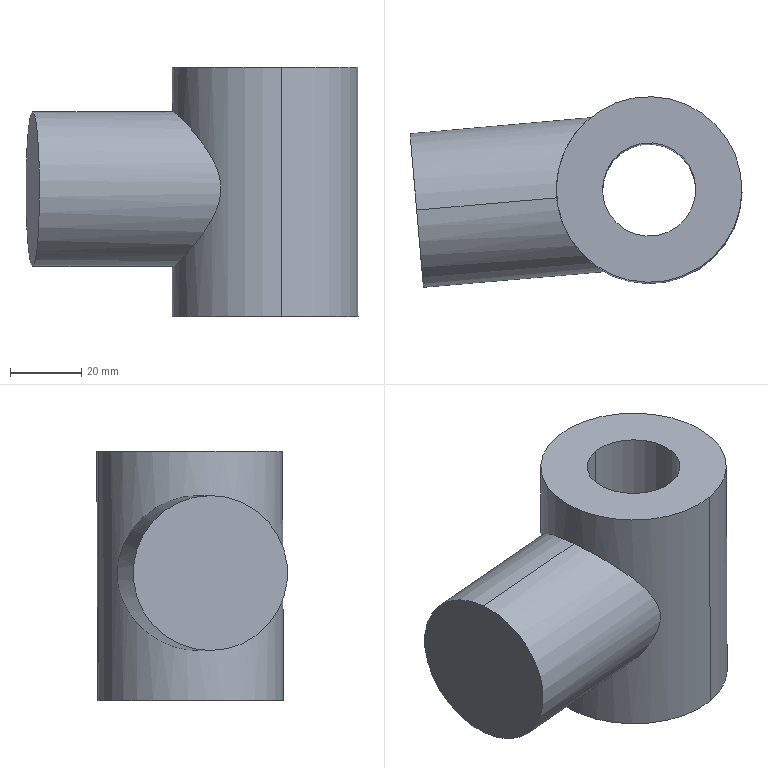Component | SolidWorks | RehabilitationChair-18-10-2 | 1 solid | 9 faces | box 93.06 x 53.47 x 70.02 mm | volume 173056 mm3 | cylinder 6 | plane 3 | commonest cylinder face diameters 43.427 x2 52.026 x2 26.129 x2
STEP:
#1=COLOUR_RGB('',0.7922,0.8196,0.9333);
#2=FILL_AREA_STYLE_COLOUR('',#1);
#3=FILL_AREA_STYLE('',(#2));
#4=SURFACE_STYLE_FILL_AREA(#3);
#5=SURFACE_SIDE_STYLE('',(#4));
#6=SURFACE_STYLE_USAGE(.BOTH.,#5);
#7=PRESENTATION_STYLE_ASSIGNMENT((#6));
#8=CARTESIAN_POINT('',(10.153,15.062,16.248));
#9=VERTEX_POINT('',#8);
#10=CARTESIAN_POINT('',(10.154,15.055,14.538));
#11=VERTEX_POINT('',#10);
#12=CARTESIAN_POINT('',(10.154,15.059,15.393));
#13=DIRECTION('',(-0.9962,-0.08716,0.));
#14=DIRECTION('',(-0.0003323,0.003798,1.));
#15=AXIS2_PLACEMENT_3D('',#12,#13,#14);
#16=CIRCLE('',#15,0.8549);
#17=EDGE_CURVE('',#9,#11,#16,.T.);
#18=ORIENTED_EDGE('',*,*,#17,.F.);
#19=CARTESIAN_POINT('',(11.698,15.197,16.248));
#20=VERTEX_POINT('',#19);
#21=CARTESIAN_POINT('',(-1.44,14.047,16.248));
#22=DIRECTION('',(0.9962,0.08716,-0.));
#23=VECTOR('',#22,39.37);
#24=LINE('',#21,#23);
#25=EDGE_CURVE('',#9,#20,#24,.T.);
#26=ORIENTED_EDGE('',*,*,#25,.T.);
#27=CARTESIAN_POINT('',(11.698,15.19,14.538));
#28=VERTEX_POINT('',#27);
#29=CARTESIAN_POINT('',(11.698,15.197,16.248));
#30=CARTESIAN_POINT('',(11.697,15.212,16.248));
#31=CARTESIAN_POINT('',(11.696,15.227,16.248));
#32=CARTESIAN_POINT('',(11.694,15.257,16.246));
#33=CARTESIAN_POINT('',(11.694,15.272,16.245));
#34=CARTESIAN_POINT('',(11.694,15.316,16.24));
#35=CARTESIAN_POINT('',(11.695,15.346,16.235));
#36=CARTESIAN_POINT('',(11.699,15.389,16.226));
#37=CARTESIAN_POINT('',(11.701,15.404,16.222));
#38=CARTESIAN_POINT('',(11.704,15.433,16.214));
#39=CARTESIAN_POINT('',(11.707,15.447,16.21));
#40=CARTESIAN_POINT('',(11.714,15.489,16.197));
#41=CARTESIAN_POINT('',(11.72,15.517,16.186));
#42=CARTESIAN_POINT('',(11.734,15.57,16.163));
#43=CARTESIAN_POINT('',(11.742,15.596,16.151));
#44=CARTESIAN_POINT('',(11.759,15.646,16.123));
#45=CARTESIAN_POINT('',(11.769,15.671,16.108));
#46=CARTESIAN_POINT('',(11.799,15.741,16.061));
#47=CARTESIAN_POINT('',(11.822,15.783,16.026));
#48=CARTESIAN_POINT('',(11.858,15.842,15.969));
#49=CARTESIAN_POINT('',(11.871,15.861,15.95));
#50=CARTESIAN_POINT('',(11.896,15.896,15.908));
#51=CARTESIAN_POINT('',(11.909,15.913,15.887));
#52=CARTESIAN_POINT('',(11.947,15.96,15.821));
#53=CARTESIAN_POINT('',(11.973,15.987,15.775));
#54=CARTESIAN_POINT('',(12.008,16.022,15.7));
#55=CARTESIAN_POINT('',(12.019,16.032,15.675));
#56=CARTESIAN_POINT('',(12.04,16.051,15.621));
#57=CARTESIAN_POINT('',(12.049,16.059,15.594));
#58=CARTESIAN_POINT('',(12.065,16.072,15.538));
#59=CARTESIAN_POINT('',(12.071,16.077,15.509));
#60=CARTESIAN_POINT('',(12.08,16.084,15.449));
#61=CARTESIAN_POINT('',(12.082,16.085,15.419));
#62=CARTESIAN_POINT('',(12.082,16.085,15.36));
#63=CARTESIAN_POINT('',(12.08,16.083,15.33));
#64=CARTESIAN_POINT('',(12.071,16.076,15.271));
#65=CARTESIAN_POINT('',(12.065,16.071,15.242));
#66=CARTESIAN_POINT('',(12.049,16.057,15.186));
#67=CARTESIAN_POINT('',(12.04,16.049,15.159));
#68=CARTESIAN_POINT('',(12.024,16.035,15.119));
#69=CARTESIAN_POINT('',(12.019,16.03,15.106));
#70=CARTESIAN_POINT('',(12.008,16.019,15.08));
#71=CARTESIAN_POINT('',(12.002,16.014,15.067));
#72=CARTESIAN_POINT('',(11.973,15.984,15.005));
#73=CARTESIAN_POINT('',(11.947,15.957,14.959));
#74=CARTESIAN_POINT('',(11.909,15.909,14.893));
#75=CARTESIAN_POINT('',(11.896,15.892,14.872));
#76=CARTESIAN_POINT('',(11.871,15.856,14.831));
#77=CARTESIAN_POINT('',(11.859,15.837,14.812));
#78=CARTESIAN_POINT('',(11.822,15.778,14.755));
#79=CARTESIAN_POINT('',(11.8,15.735,14.721));
#80=CARTESIAN_POINT('',(11.774,15.677,14.682));
#81=CARTESIAN_POINT('',(11.769,15.665,14.675));
#82=CARTESIAN_POINT('',(11.76,15.641,14.66));
#83=CARTESIAN_POINT('',(11.755,15.628,14.653));
#84=CARTESIAN_POINT('',(11.742,15.59,14.632));
#85=CARTESIAN_POINT('',(11.734,15.564,14.62));
#86=CARTESIAN_POINT('',(11.72,15.511,14.598));
#87=CARTESIAN_POINT('',(11.715,15.483,14.587));
#88=CARTESIAN_POINT('',(11.705,15.427,14.57));
#89=CARTESIAN_POINT('',(11.701,15.398,14.562));
#90=CARTESIAN_POINT('',(11.693,15.31,14.544));
#91=CARTESIAN_POINT('',(11.693,15.251,14.538));
#92=CARTESIAN_POINT('',(11.698,15.19,14.538));
#93=B_SPLINE_CURVE_WITH_KNOTS('',3,(#29,#30,#31,#32,#33,#34,#35,#36,#37,#38,#39,#40,#41,#42,#43,#44,#45,#46,#47,#48,#49,#50,#51,#52,#53,#54,#55,#56,#57,#58,#59,#60,#61,#62,#63,#64,#65,#66,#67,#68,#69,#70,#71,#72,#73,#74,#75,#76,#77,#78,#79,#80,#81,#82,#83,#84,#85,#86,#87,#88,#89,#90,#91,#92),.UNSPECIFIED.,.F.,.F.,(4,2,2,2,2,2,2,2,2,2,2,2,2,2,2,2,2,2,2,2,2,2,2,2,2,2,2,2,2,2,2,4),(0.07253,0.07367,0.0748,0.07706,0.07819,0.07933,0.08159,0.08385,0.08612,0.09065,0.09291,0.09517,0.0997,0.102,0.1042,0.1065,0.1088,0.111,0.1133,0.1155,0.1167,0.1178,0.1223,0.1246,0.1269,0.1314,0.1325,0.1337,0.1359,0.1382,0.1405,0.145),.UNSPECIFIED.);
#94=EDGE_CURVE('',#20,#28,#93,.T.);
#95=ORIENTED_EDGE('',*,*,#94,.T.);
#96=CARTESIAN_POINT('',(-1.44,14.041,14.538));
#97=DIRECTION('',(0.9962,0.08716,-0.));
#98=VECTOR('',#97,39.37);
#99=LINE('',#96,#98);
#100=EDGE_CURVE('',#11,#28,#99,.T.);
#101=ORIENTED_EDGE('',*,*,#100,.F.);
#102=EDGE_LOOP('',(#18,#26,#95,#101));
#103=FACE_OUTER_BOUND('',#102,.T.);
#104=CARTESIAN_POINT('',(-1.44,14.044,15.393));
#105=DIRECTION('',(0.9962,0.08716,-0.));
#106=DIRECTION('',(0.0003323,-0.003798,-1.));
#107=AXIS2_PLACEMENT_3D('',#104,#105,#106);
#108=CYLINDRICAL_SURFACE('',#107,0.8549);
#109=ADVANCED_FACE('',(#103),#108,.T.);
#110=CARTESIAN_POINT('',(12.897,14.269,13.99));
#111=VERTEX_POINT('',#110);
#112=CARTESIAN_POINT('',(12.541,16.286,13.982));
#113=VERTEX_POINT('',#112);
#114=CARTESIAN_POINT('',(12.719,15.278,13.986));
#115=DIRECTION('',(-0.0003323,0.003798,1.));
#116=DIRECTION('',(-0.9962,-0.08716,0.));
#117=AXIS2_PLACEMENT_3D('',#114,#115,#116);
#118=CIRCLE('',#117,1.024);
#119=EDGE_CURVE('',#111,#113,#118,.T.);
#120=ORIENTED_EDGE('',*,*,#119,.T.);
#121=CARTESIAN_POINT('',(12.54,16.297,16.731));
#122=VERTEX_POINT('',#121);
#123=CARTESIAN_POINT('',(12.541,16.283,13.195));
#124=DIRECTION('',(-0.0003323,0.003798,1.));
#125=VECTOR('',#124,39.37);
#126=LINE('',#123,#125);
#127=EDGE_CURVE('',#113,#122,#126,.T.);
#128=ORIENTED_EDGE('',*,*,#127,.T.);
#129=CARTESIAN_POINT('',(12.896,14.279,16.739));
#130=VERTEX_POINT('',#129);
#131=CARTESIAN_POINT('',(12.718,15.288,16.735));
#132=DIRECTION('',(-0.0003323,0.003798,1.));
#133=DIRECTION('',(-0.9962,-0.08716,0.));
#134=AXIS2_PLACEMENT_3D('',#131,#132,#133);
#135=CIRCLE('',#134,1.024);
#136=EDGE_CURVE('',#130,#122,#135,.T.);
#137=ORIENTED_EDGE('',*,*,#136,.F.);
#138=CARTESIAN_POINT('',(12.897,14.266,13.203));
#139=DIRECTION('',(-0.0003323,0.003798,1.));
#140=VECTOR('',#139,39.37);
#141=LINE('',#138,#140);
#142=EDGE_CURVE('',#111,#130,#141,.T.);
#143=ORIENTED_EDGE('',*,*,#142,.F.);
#144=EDGE_LOOP('',(#120,#128,#137,#143));
#145=FACE_OUTER_BOUND('',#144,.T.);
#146=CARTESIAN_POINT('',(12.719,15.275,13.199));
#147=DIRECTION('',(-0.0003323,0.003798,1.));
#148=DIRECTION('',(0.1736,-0.9848,0.003798));
#149=AXIS2_PLACEMENT_3D('',#146,#147,#148);
#150=CYLINDRICAL_SURFACE('',#149,1.024);
#151=ADVANCED_FACE('',(#145),#150,.T.);
#152=CARTESIAN_POINT('',(12.629,15.795,16.733));
#153=VERTEX_POINT('',#152);
#154=CARTESIAN_POINT('',(12.807,14.781,16.737));
#155=VERTEX_POINT('',#154);
#156=CARTESIAN_POINT('',(12.718,15.288,16.735));
#157=DIRECTION('',(-0.0003323,0.003798,1.));
#158=DIRECTION('',(0.1736,-0.9848,0.003798));
#159=AXIS2_PLACEMENT_3D('',#156,#157,#158);
#160=CIRCLE('',#159,0.5144);
#161=EDGE_CURVE('',#153,#155,#160,.T.);
#162=ORIENTED_EDGE('',*,*,#161,.T.);
#163=CARTESIAN_POINT('',(12.808,14.771,13.988));
#164=VERTEX_POINT('',#163);
#165=CARTESIAN_POINT('',(12.807,14.781,16.734));
#166=DIRECTION('',(0.0003323,-0.003798,-1.));
#167=VECTOR('',#166,39.37);
#168=LINE('',#165,#167);
#169=EDGE_CURVE('',#155,#164,#168,.T.);
#170=ORIENTED_EDGE('',*,*,#169,.T.);
#171=CARTESIAN_POINT('',(12.63,15.784,13.984));
#172=VERTEX_POINT('',#171);
#173=CARTESIAN_POINT('',(12.719,15.278,13.986));
#174=DIRECTION('',(0.0003323,-0.003798,-1.));
#175=DIRECTION('',(0.1736,-0.9848,0.003798));
#176=AXIS2_PLACEMENT_3D('',#173,#174,#175);
#177=CIRCLE('',#176,0.5144);
#178=EDGE_CURVE('',#164,#172,#177,.T.);
#179=ORIENTED_EDGE('',*,*,#178,.T.);
#180=CARTESIAN_POINT('',(12.629,15.795,16.73));
#181=DIRECTION('',(0.0003323,-0.003798,-1.));
#182=VECTOR('',#181,39.37);
#183=LINE('',#180,#182);
#184=EDGE_CURVE('',#153,#172,#183,.T.);
#185=ORIENTED_EDGE('',*,*,#184,.F.);
#186=EDGE_LOOP('',(#162,#170,#179,#185));
#187=FACE_OUTER_BOUND('',#186,.T.);
#188=CARTESIAN_POINT('',(12.718,15.288,16.732));
#189=DIRECTION('',(0.0003323,-0.003798,-1.));
#190=DIRECTION('',(-0.1736,0.9848,-0.003798));
#191=AXIS2_PLACEMENT_3D('',#188,#189,#190);
#192=CYLINDRICAL_SURFACE('',#191,0.5144);
#193=ADVANCED_FACE('',(#187),#192,.F.);
#194=ORIENTED_EDGE('',*,*,#119,.F.);
#195=CARTESIAN_POINT('',(12.719,15.278,13.986));
#196=DIRECTION('',(-0.0003323,0.003798,1.));
#197=DIRECTION('',(-0.9962,-0.08716,0.));
#198=AXIS2_PLACEMENT_3D('',#195,#196,#197);
#199=CIRCLE('',#198,1.024);
#200=EDGE_CURVE('',#113,#111,#199,.T.);
#201=ORIENTED_EDGE('',*,*,#200,.F.);
#202=EDGE_LOOP('',(#194,#201));
#203=FACE_OUTER_BOUND('',#202,.T.);
#204=CARTESIAN_POINT('',(12.719,15.278,13.986));
#205=DIRECTION('',(0.0003323,-0.003798,-1.));
#206=DIRECTION('',(0.1736,-0.9848,0.003798));
#207=AXIS2_PLACEMENT_3D('',#204,#205,#206);
#208=CIRCLE('',#207,0.5144);
#209=EDGE_CURVE('',#172,#164,#208,.T.);
#210=ORIENTED_EDGE('',*,*,#209,.F.);
#211=ORIENTED_EDGE('',*,*,#178,.F.);
#212=EDGE_LOOP('',(#210,#211));
#213=FACE_BOUND('',#212,.T.);
#214=CARTESIAN_POINT('',(13.727,15.455,13.986));
#215=DIRECTION('',(-0.0003323,0.003798,1.));
#216=DIRECTION('',(0.1736,-0.9848,0.003798));
#217=AXIS2_PLACEMENT_3D('',#214,#215,#216);
#218=PLANE('',#217);
#219=ADVANCED_FACE('',(#203,#213),#218,.F.);
#220=CARTESIAN_POINT('',(10.154,15.059,15.393));
#221=DIRECTION('',(-0.9962,-0.08716,0.));
#222=DIRECTION('',(-0.0003323,0.003798,1.));
#223=AXIS2_PLACEMENT_3D('',#220,#221,#222);
#224=CIRCLE('',#223,0.8549);
#225=EDGE_CURVE('',#11,#9,#224,.T.);
#226=ORIENTED_EDGE('',*,*,#225,.T.);
#227=ORIENTED_EDGE('',*,*,#17,.T.);
#228=EDGE_LOOP('',(#226,#227));
#229=FACE_OUTER_BOUND('',#228,.T.);
#230=CARTESIAN_POINT('',(9.938,17.521,42.747));
#231=DIRECTION('',(-0.9962,-0.08716,0.));
#232=DIRECTION('',(-0.0003323,0.003798,1.));
#233=AXIS2_PLACEMENT_3D('',#230,#231,#232);
#234=PLANE('',#233);
#235=ADVANCED_FACE('',(#229),#234,.T.);
#236=ORIENTED_EDGE('',*,*,#25,.F.);
#237=ORIENTED_EDGE('',*,*,#225,.F.);
#238=ORIENTED_EDGE('',*,*,#100,.T.);
#239=CARTESIAN_POINT('',(11.698,15.19,14.538));
#240=CARTESIAN_POINT('',(11.704,15.13,14.539));
#241=CARTESIAN_POINT('',(11.714,15.072,14.545));
#242=CARTESIAN_POINT('',(11.733,15.001,14.561));
#243=CARTESIAN_POINT('',(11.737,14.987,14.564));
#244=CARTESIAN_POINT('',(11.746,14.96,14.572));
#245=CARTESIAN_POINT('',(11.75,14.946,14.576));
#246=CARTESIAN_POINT('',(11.765,14.905,14.59));
#247=CARTESIAN_POINT('',(11.776,14.879,14.6));
#248=CARTESIAN_POINT('',(11.799,14.829,14.623));
#249=CARTESIAN_POINT('',(11.811,14.805,14.635));
#250=CARTESIAN_POINT('',(11.837,14.759,14.663));
#251=CARTESIAN_POINT('',(11.851,14.736,14.678));
#252=CARTESIAN_POINT('',(11.893,14.672,14.725));
#253=CARTESIAN_POINT('',(11.923,14.634,14.76));
#254=CARTESIAN_POINT('',(11.968,14.583,14.817));
#255=CARTESIAN_POINT('',(11.984,14.567,14.836));
#256=CARTESIAN_POINT('',(12.015,14.536,14.878));
#257=CARTESIAN_POINT('',(12.031,14.522,14.899));
#258=CARTESIAN_POINT('',(12.077,14.482,14.965));
#259=CARTESIAN_POINT('',(12.106,14.46,15.011));
#260=CARTESIAN_POINT('',(12.14,14.436,15.073));
#261=CARTESIAN_POINT('',(12.147,14.432,15.086));
#262=CARTESIAN_POINT('',(12.16,14.424,15.112));
#263=CARTESIAN_POINT('',(12.166,14.42,15.125));
#264=CARTESIAN_POINT('',(12.184,14.409,15.165));
#265=CARTESIAN_POINT('',(12.194,14.402,15.193));
#266=CARTESIAN_POINT('',(12.207,14.395,15.235));
#267=CARTESIAN_POINT('',(12.211,14.393,15.249));
#268=CARTESIAN_POINT('',(12.218,14.389,15.278));
#269=CARTESIAN_POINT('',(12.221,14.387,15.293));
#270=CARTESIAN_POINT('',(12.229,14.383,15.337));
#271=CARTESIAN_POINT('',(12.231,14.382,15.367));
#272=CARTESIAN_POINT('',(12.231,14.382,15.427));
#273=CARTESIAN_POINT('',(12.229,14.384,15.456));
#274=CARTESIAN_POINT('',(12.219,14.389,15.516));
#275=CARTESIAN_POINT('',(12.211,14.394,15.545));
#276=CARTESIAN_POINT('',(12.194,14.404,15.601));
#277=CARTESIAN_POINT('',(12.183,14.41,15.628));
#278=CARTESIAN_POINT('',(12.165,14.422,15.668));
#279=CARTESIAN_POINT('',(12.159,14.426,15.681));
#280=CARTESIAN_POINT('',(12.146,14.434,15.707));
#281=CARTESIAN_POINT('',(12.14,14.439,15.719));
#282=CARTESIAN_POINT('',(12.106,14.463,15.782));
#283=CARTESIAN_POINT('',(12.076,14.486,15.828));
#284=CARTESIAN_POINT('',(12.03,14.526,15.893));
#285=CARTESIAN_POINT('',(12.014,14.541,15.914));
#286=CARTESIAN_POINT('',(11.983,14.572,15.955));
#287=CARTESIAN_POINT('',(11.968,14.588,15.975));
#288=CARTESIAN_POINT('',(11.922,14.64,16.031));
#289=CARTESIAN_POINT('',(11.892,14.678,16.066));
#290=CARTESIAN_POINT('',(11.85,14.742,16.112));
#291=CARTESIAN_POINT('',(11.836,14.765,16.127));
#292=CARTESIAN_POINT('',(11.81,14.812,16.154));
#293=CARTESIAN_POINT('',(11.798,14.836,16.167));
#294=CARTESIAN_POINT('',(11.775,14.886,16.189));
#295=CARTESIAN_POINT('',(11.764,14.912,16.199));
#296=CARTESIAN_POINT('',(11.745,14.966,16.217));
#297=CARTESIAN_POINT('',(11.736,14.994,16.224));
#298=CARTESIAN_POINT('',(11.713,15.079,16.242));
#299=CARTESIAN_POINT('',(11.703,15.137,16.248));
#300=CARTESIAN_POINT('',(11.698,15.197,16.248));
#301=B_SPLINE_CURVE_WITH_KNOTS('',3,(#239,#240,#241,#242,#243,#244,#245,#246,#247,#248,#249,#250,#251,#252,#253,#254,#255,#256,#257,#258,#259,#260,#261,#262,#263,#264,#265,#266,#267,#268,#269,#270,#271,#272,#273,#274,#275,#276,#277,#278,#279,#280,#281,#282,#283,#284,#285,#286,#287,#288,#289,#290,#291,#292,#293,#294,#295,#296,#297,#298,#299,#300),.UNSPECIFIED.,.F.,.F.,(4,2,2,2,2,2,2,2,2,2,2,2,2,2,2,2,2,2,2,2,2,2,2,2,2,2,2,2,2,2,4),(0.,0.004533,0.005667,0.0068,0.009067,0.01133,0.0136,0.01813,0.0204,0.02267,0.0272,0.02833,0.02947,0.03173,0.03287,0.034,0.03627,0.03853,0.0408,0.04307,0.0442,0.04533,0.04987,0.05213,0.0544,0.05893,0.0612,0.06347,0.06573,0.068,0.07253),.UNSPECIFIED.);
#302=EDGE_CURVE('',#28,#20,#301,.T.);
#303=ORIENTED_EDGE('',*,*,#302,.T.);
#304=EDGE_LOOP('',(#236,#237,#238,#303));
#305=FACE_OUTER_BOUND('',#304,.T.);
#306=CARTESIAN_POINT('',(-1.44,14.044,15.393));
#307=DIRECTION('',(0.9962,0.08716,-0.));
#308=DIRECTION('',(0.0003323,-0.003798,-1.));
#309=AXIS2_PLACEMENT_3D('',#306,#307,#308);
#310=CYLINDRICAL_SURFACE('',#309,0.8549);
#311=ADVANCED_FACE('',(#305),#310,.T.);
#312=ORIENTED_EDGE('',*,*,#161,.F.);
#313=CARTESIAN_POINT('',(12.718,15.288,16.735));
#314=DIRECTION('',(-0.0003323,0.003798,1.));
#315=DIRECTION('',(0.1736,-0.9848,0.003798));
#316=AXIS2_PLACEMENT_3D('',#313,#314,#315);
#317=CIRCLE('',#316,0.5144);
#318=EDGE_CURVE('',#155,#153,#317,.T.);
#319=ORIENTED_EDGE('',*,*,#318,.F.);
#320=EDGE_LOOP('',(#312,#319));
#321=FACE_BOUND('',#320,.T.);
#322=ORIENTED_EDGE('',*,*,#136,.T.);
#323=CARTESIAN_POINT('',(12.718,15.288,16.735));
#324=DIRECTION('',(-0.0003323,0.003798,1.));
#325=DIRECTION('',(-0.9962,-0.08716,0.));
#326=AXIS2_PLACEMENT_3D('',#323,#324,#325);
#327=CIRCLE('',#326,1.024);
#328=EDGE_CURVE('',#122,#130,#327,.T.);
#329=ORIENTED_EDGE('',*,*,#328,.T.);
#330=EDGE_LOOP('',(#322,#329));
#331=FACE_OUTER_BOUND('',#330,.T.);
#332=CARTESIAN_POINT('',(12.718,15.288,16.735));
#333=DIRECTION('',(-0.0003323,0.003798,1.));
#334=DIRECTION('',(0.9962,0.08716,-0.));
#335=AXIS2_PLACEMENT_3D('',#332,#333,#334);
#336=PLANE('',#335);
#337=ADVANCED_FACE('',(#321,#331),#336,.T.);
#338=ORIENTED_EDGE('',*,*,#127,.F.);
#339=ORIENTED_EDGE('',*,*,#200,.T.);
#340=ORIENTED_EDGE('',*,*,#142,.T.);
#341=ORIENTED_EDGE('',*,*,#328,.F.);
#342=EDGE_LOOP('',(#338,#339,#340,#341));
#343=FACE_OUTER_BOUND('',#342,.T.);
#344=ORIENTED_EDGE('',*,*,#302,.F.);
#345=ORIENTED_EDGE('',*,*,#94,.F.);
#346=EDGE_LOOP('',(#344,#345));
#347=FACE_BOUND('',#346,.T.);
#348=CARTESIAN_POINT('',(12.719,15.275,13.199));
#349=DIRECTION('',(-0.0003323,0.003798,1.));
#350=DIRECTION('',(0.1736,-0.9848,0.003798));
#351=AXIS2_PLACEMENT_3D('',#348,#349,#350);
#352=CYLINDRICAL_SURFACE('',#351,1.024);
#353=ADVANCED_FACE('',(#343,#347),#352,.T.);
#354=ORIENTED_EDGE('',*,*,#169,.F.);
#355=ORIENTED_EDGE('',*,*,#318,.T.);
#356=ORIENTED_EDGE('',*,*,#184,.T.);
#357=ORIENTED_EDGE('',*,*,#209,.T.);
#358=EDGE_LOOP('',(#354,#355,#356,#357));
#359=FACE_OUTER_BOUND('',#358,.T.);
#360=CARTESIAN_POINT('',(12.718,15.288,16.732));
#361=DIRECTION('',(0.0003323,-0.003798,-1.));
#362=DIRECTION('',(-0.1736,0.9848,-0.003798));
#363=AXIS2_PLACEMENT_3D('',#360,#361,#362);
#364=CYLINDRICAL_SURFACE('',#363,0.5144);
#365=ADVANCED_FACE('',(#359),#364,.F.);
#366=CLOSED_SHELL('',(#109,#151,#193,#219,#235,#311,#337,#353,#365));
#367=MANIFOLD_SOLID_BREP('',#366);
#368=STYLED_ITEM('',(#7),#367);
#369=(LENGTH_UNIT()NAMED_UNIT(*)SI_UNIT($,.METRE.));
#370=LENGTH_MEASURE_WITH_UNIT(LENGTH_MEASURE(0.0254),#369);
#371=DIMENSIONAL_EXPONENTS(1.,0.,0.,0.,0.,0.,0.);
#372=(CONVERSION_BASED_UNIT('',#370)LENGTH_UNIT()NAMED_UNIT(#371));
#373=UNCERTAINTY_MEASURE_WITH_UNIT(LENGTH_MEASURE(0.00001),#372,'','');
#374=(NAMED_UNIT(*)PLANE_ANGLE_UNIT()SI_UNIT($,.RADIAN.));
#375=(NAMED_UNIT(*)SI_UNIT($,.STERADIAN.)SOLID_ANGLE_UNIT());
#376=(GEOMETRIC_REPRESENTATION_CONTEXT(3)GLOBAL_UNCERTAINTY_ASSIGNED_CONTEXT((#373))GLOBAL_UNIT_ASSIGNED_CONTEXT((#372,#374,#375))REPRESENTATION_CONTEXT('',''));
#377=MECHANICAL_DESIGN_GEOMETRIC_PRESENTATION_REPRESENTATION('',(#368),#376);
#378=CARTESIAN_POINT('',(0.,0.,0.));
#379=DIRECTION('',(0.,0.,1.));
#380=DIRECTION('',(1.,0.,0.));
#381=AXIS2_PLACEMENT_3D('',#378,#379,#380);
#382=(LENGTH_UNIT()NAMED_UNIT(*)SI_UNIT($,.METRE.));
#383=LENGTH_MEASURE_WITH_UNIT(LENGTH_MEASURE(0.0254),#382);
#384=DIMENSIONAL_EXPONENTS(1.,0.,0.,0.,0.,0.,0.);
#385=(CONVERSION_BASED_UNIT('',#383)LENGTH_UNIT()NAMED_UNIT(#384));
#386=UNCERTAINTY_MEASURE_WITH_UNIT(LENGTH_MEASURE(0.00001),#385,'','');
#387=(NAMED_UNIT(*)PLANE_ANGLE_UNIT()SI_UNIT($,.RADIAN.));
#388=(NAMED_UNIT(*)SI_UNIT($,.STERADIAN.)SOLID_ANGLE_UNIT());
#389=(GEOMETRIC_REPRESENTATION_CONTEXT(3)GLOBAL_UNCERTAINTY_ASSIGNED_CONTEXT((#386))GLOBAL_UNIT_ASSIGNED_CONTEXT((#385,#387,#388))REPRESENTATION_CONTEXT('',''));
#390=ADVANCED_BREP_SHAPE_REPRESENTATION('',(#367,#381),#389);
#391=PRESENTATION_LAYER_ASSIGNMENT('','',(#368));